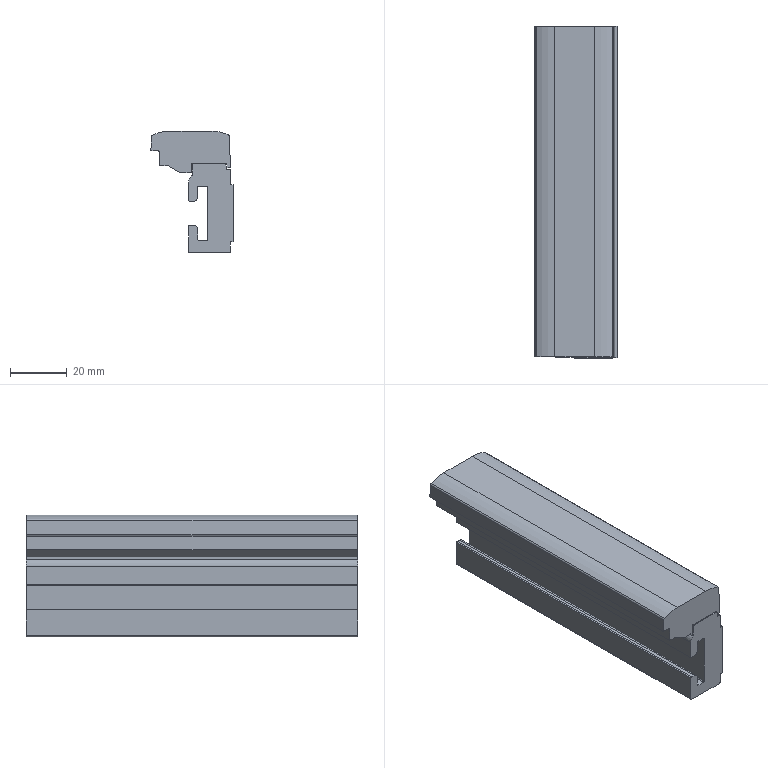Component | SolidWorks | DGC-18-280-G-PPV-A-1_532446 DGC-18-G-PG---(SG)_1-1 | 1 solid | 74 faces | volume 81466 mm3 | plane 37 | cylinder 29 | cone 8 | commonest cylinder face diameters 0.6 x5 1 x5 4.134 x4 3 x4 0.4 x3 2 x2 30 x2 1.2 x2